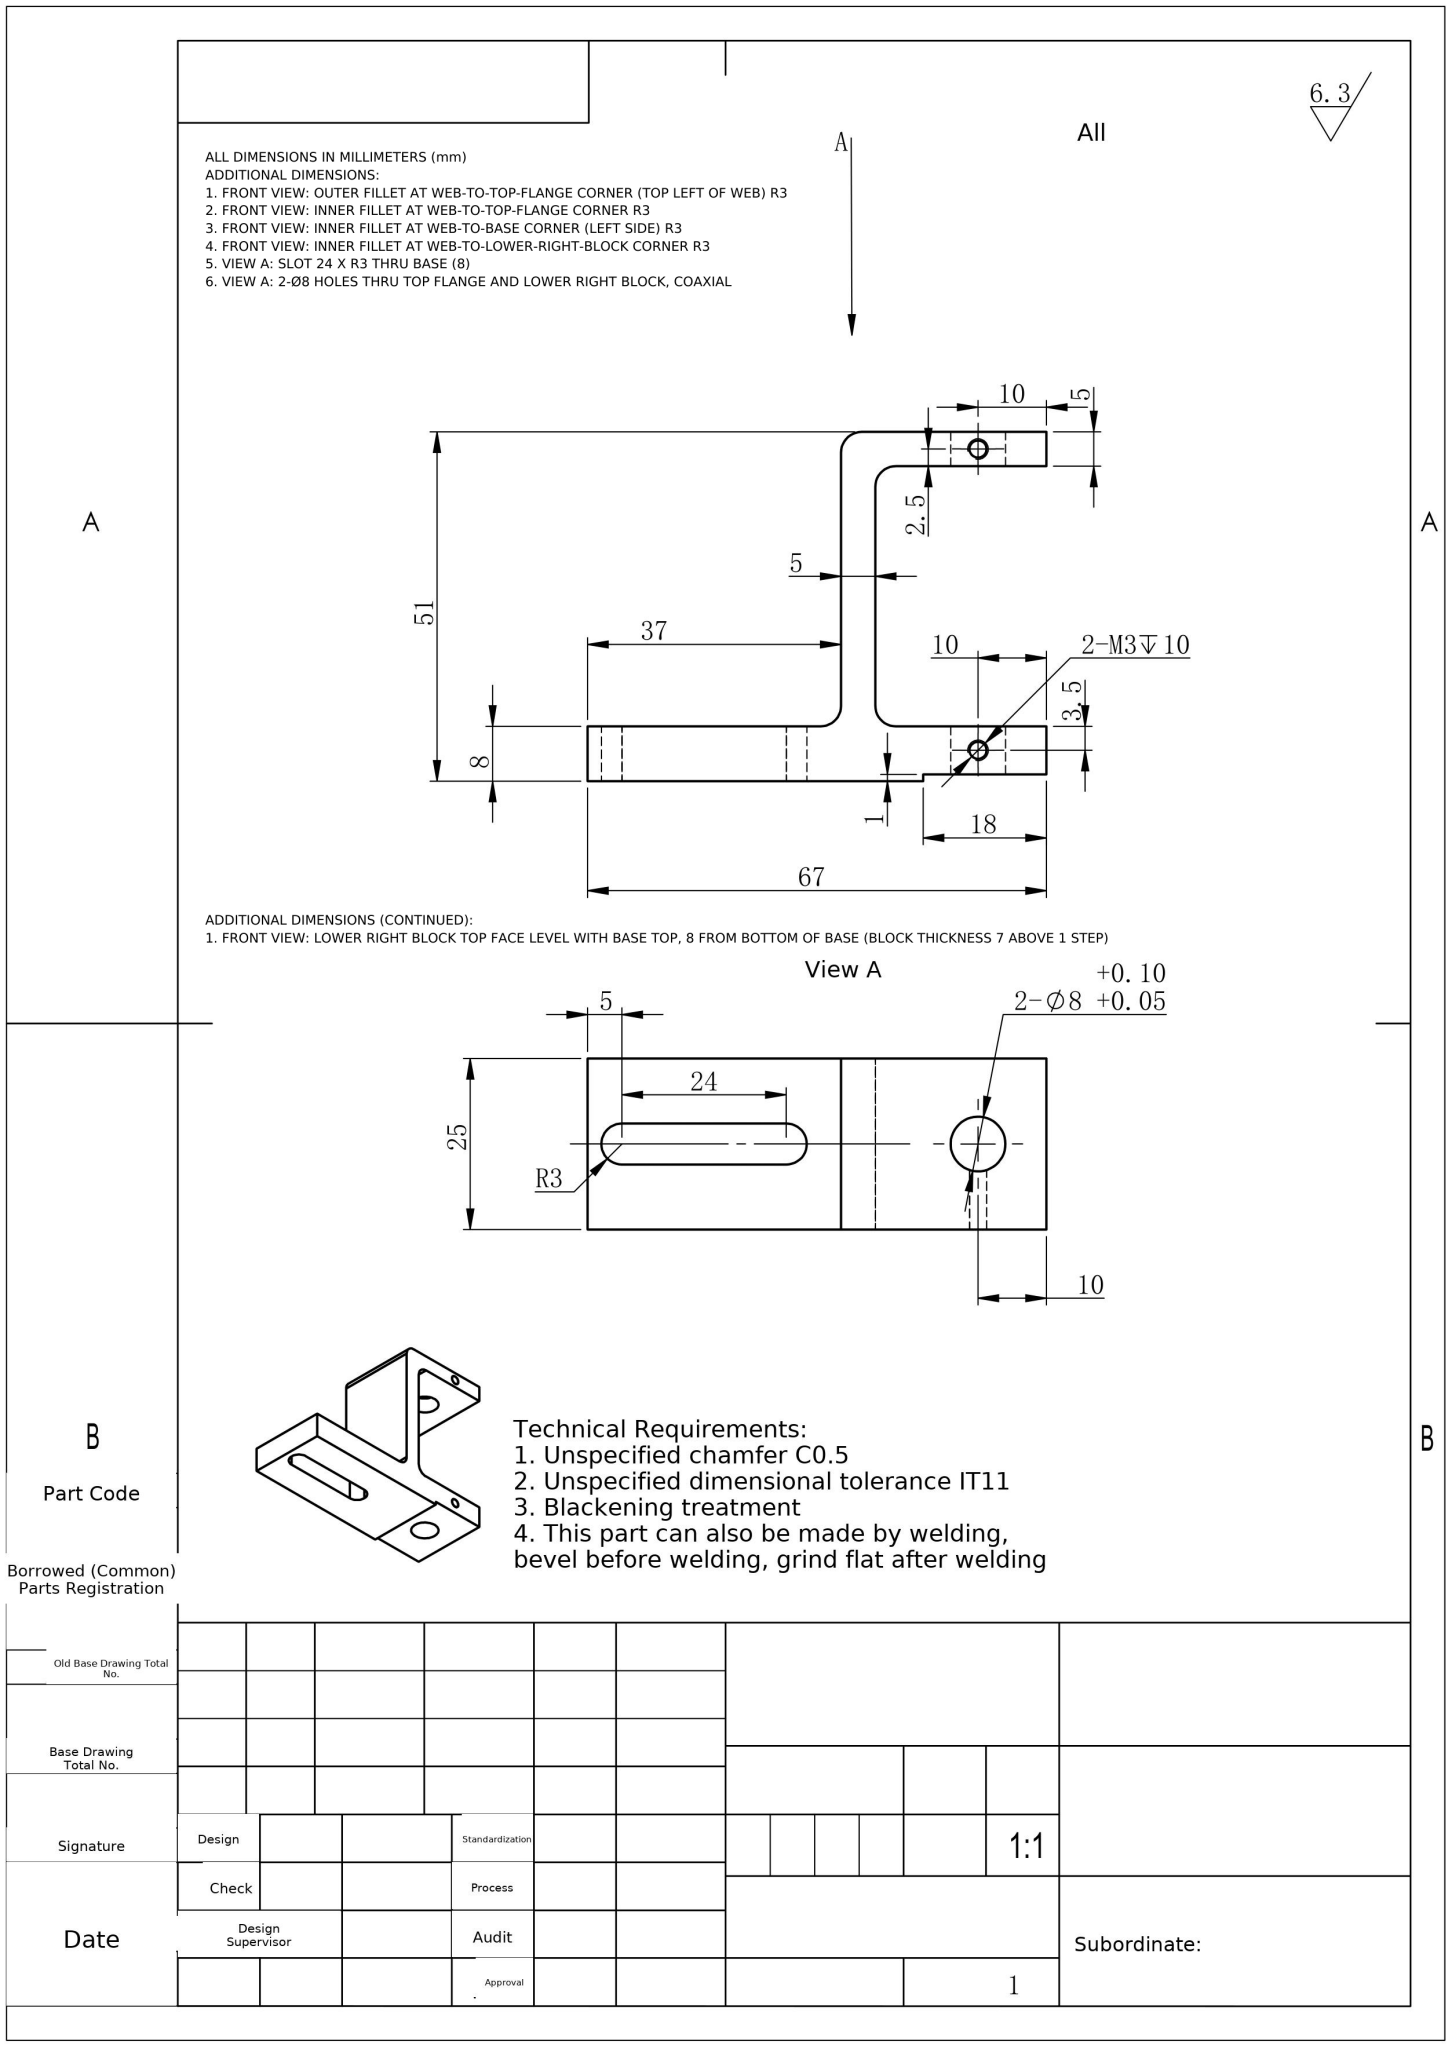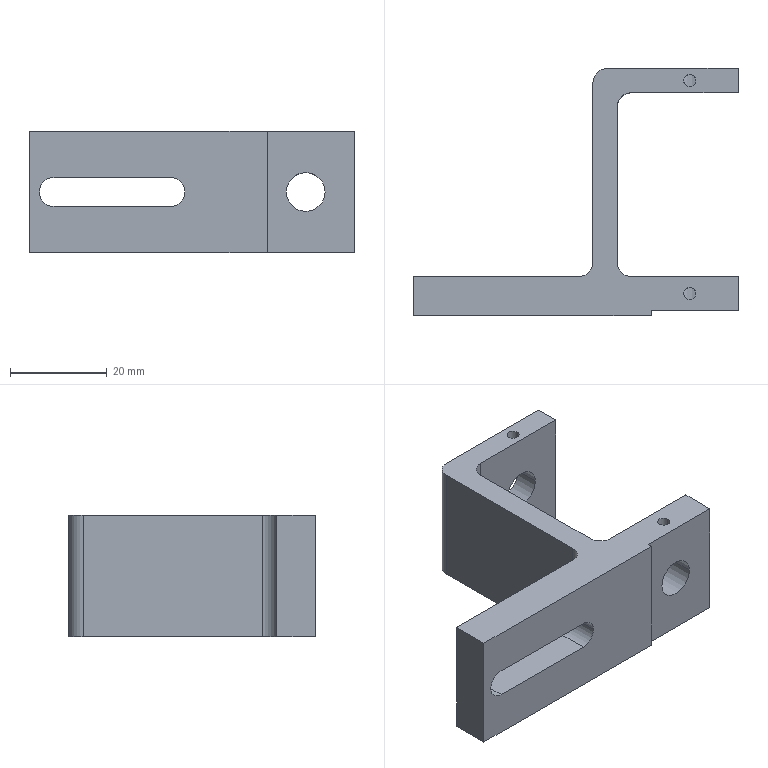Part | NX | mm | 1 solid | 32 faces | box 67 x 51 x 25 mm | volume 19481 mm3 | cylinder 16 | plane 16 | commonest cylinder face diameters 6 x8 2.5 x4 8 x4